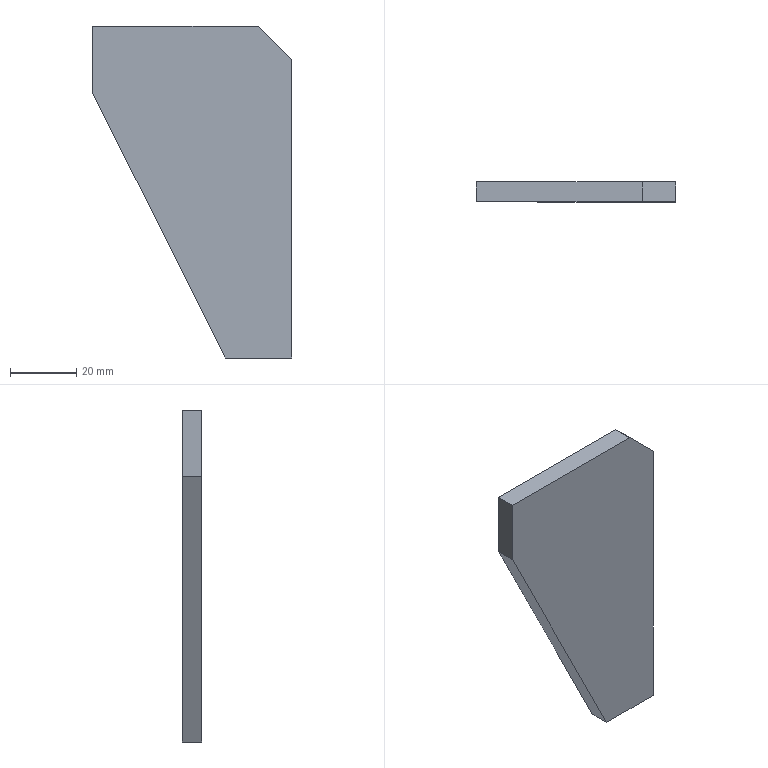Component | SolidWorks | JHK-B1004Stiffener-3 | 1 solid | 8 faces | box 60 x 6 x 100 mm | volume 26100 mm3 | plane 8 | material Q235A
build123d program:
from build123d import *

# Parameters (mm, degrees)
BOSS_EXTRUDE1_DEPTH = 3
CHAMFER1_SIZE       = 10


with BuildPart() as part:
    # Sketch1 → Boss-Extrude1 (new, symmetric)
    with BuildSketch(Plane(origin=(0, 0, 0), x_dir=(0, 0, -1), z_dir=(0, 1, 0))):
        Polygon((0, 60), (0, 0), (100, 0), (100, 20), (20, 60), align=None)
    extrude(amount=BOSS_EXTRUDE1_DEPTH, both=True)

    # Chamfer1
    chamfer1_edges = [part.edges().sort_by_distance(p)[0] for p in [
        (0, 0, 0),
    ]]
    chamfer(chamfer1_edges, length=CHAMFER1_SIZE)


solid = part.part

# Placed as in the assembly
solid = solid.moved(Location((270, -125, -261), (0, 0, 0)))
STEP:
#1=COLOUR_RGB('',0.7922,0.8196,0.9333);
#2=FILL_AREA_STYLE_COLOUR('',#1);
#3=FILL_AREA_STYLE('',(#2));
#4=SURFACE_STYLE_FILL_AREA(#3);
#5=SURFACE_SIDE_STYLE('',(#4));
#6=SURFACE_STYLE_USAGE(.BOTH.,#5);
#7=PRESENTATION_STYLE_ASSIGNMENT((#6));
#8=CARTESIAN_POINT('',(10.63,-4.803,-10.669));
#9=VERTEX_POINT('',#8);
#10=CARTESIAN_POINT('',(10.63,-4.803,-14.213));
#11=VERTEX_POINT('',#10);
#12=CARTESIAN_POINT('',(10.63,-4.803,-10.276));
#13=DIRECTION('',(0.,0.,-1.));
#14=VECTOR('',#13,39.37);
#15=LINE('',#12,#14);
#16=EDGE_CURVE('',#9,#11,#15,.T.);
#17=ORIENTED_EDGE('',*,*,#16,.F.);
#18=CARTESIAN_POINT('',(10.63,-5.039,-10.669));
#19=VERTEX_POINT('',#18);
#20=CARTESIAN_POINT('',(10.63,-4.803,-10.669));
#21=DIRECTION('',(0.,-1.,0.));
#22=VECTOR('',#21,39.37);
#23=LINE('',#20,#22);
#24=EDGE_CURVE('',#9,#19,#23,.T.);
#25=ORIENTED_EDGE('',*,*,#24,.T.);
#26=CARTESIAN_POINT('',(10.63,-5.039,-14.213));
#27=VERTEX_POINT('',#26);
#28=CARTESIAN_POINT('',(10.63,-5.039,-10.276));
#29=DIRECTION('',(0.,0.,-1.));
#30=VECTOR('',#29,39.37);
#31=LINE('',#28,#30);
#32=EDGE_CURVE('',#19,#27,#31,.T.);
#33=ORIENTED_EDGE('',*,*,#32,.T.);
#34=CARTESIAN_POINT('',(10.63,-4.803,-14.213));
#35=DIRECTION('',(0.,-1.,0.));
#36=VECTOR('',#35,39.37);
#37=LINE('',#34,#36);
#38=EDGE_CURVE('',#11,#27,#37,.T.);
#39=ORIENTED_EDGE('',*,*,#38,.F.);
#40=EDGE_LOOP('',(#17,#25,#33,#39));
#41=FACE_OUTER_BOUND('',#40,.T.);
#42=CARTESIAN_POINT('',(10.63,-4.803,-10.276));
#43=DIRECTION('',(-1.,0.,0.));
#44=DIRECTION('',(0.,0.,1.));
#45=AXIS2_PLACEMENT_3D('',#42,#43,#44);
#46=PLANE('',#45);
#47=ADVANCED_FACE('',(#41),#46,.F.);
#48=CARTESIAN_POINT('',(9.843,-5.039,-14.213));
#49=VERTEX_POINT('',#48);
#50=CARTESIAN_POINT('',(10.63,-5.039,-14.213));
#51=DIRECTION('',(-1.,0.,0.));
#52=VECTOR('',#51,39.37);
#53=LINE('',#50,#52);
#54=EDGE_CURVE('',#27,#49,#53,.T.);
#55=ORIENTED_EDGE('',*,*,#54,.T.);
#56=CARTESIAN_POINT('',(9.843,-4.803,-14.213));
#57=VERTEX_POINT('',#56);
#58=CARTESIAN_POINT('',(9.843,-4.803,-14.213));
#59=DIRECTION('',(0.,-1.,0.));
#60=VECTOR('',#59,39.37);
#61=LINE('',#58,#60);
#62=EDGE_CURVE('',#57,#49,#61,.T.);
#63=ORIENTED_EDGE('',*,*,#62,.F.);
#64=CARTESIAN_POINT('',(10.63,-4.803,-14.213));
#65=DIRECTION('',(-1.,0.,0.));
#66=VECTOR('',#65,39.37);
#67=LINE('',#64,#66);
#68=EDGE_CURVE('',#11,#57,#67,.T.);
#69=ORIENTED_EDGE('',*,*,#68,.F.);
#70=ORIENTED_EDGE('',*,*,#38,.T.);
#71=EDGE_LOOP('',(#55,#63,#69,#70));
#72=FACE_OUTER_BOUND('',#71,.T.);
#73=CARTESIAN_POINT('',(10.63,-4.803,-14.213));
#74=DIRECTION('',(0.,0.,1.));
#75=DIRECTION('',(1.,0.,0.));
#76=AXIS2_PLACEMENT_3D('',#73,#74,#75);
#77=PLANE('',#76);
#78=ADVANCED_FACE('',(#72),#77,.F.);
#79=CARTESIAN_POINT('',(8.268,-5.039,-11.063));
#80=VERTEX_POINT('',#79);
#81=CARTESIAN_POINT('',(9.843,-5.039,-14.213));
#82=DIRECTION('',(-0.4472,0.,0.8944));
#83=VECTOR('',#82,39.37);
#84=LINE('',#81,#83);
#85=EDGE_CURVE('',#49,#80,#84,.T.);
#86=ORIENTED_EDGE('',*,*,#85,.T.);
#87=CARTESIAN_POINT('',(8.268,-4.803,-11.063));
#88=VERTEX_POINT('',#87);
#89=CARTESIAN_POINT('',(8.268,-4.803,-11.063));
#90=DIRECTION('',(0.,-1.,0.));
#91=VECTOR('',#90,39.37);
#92=LINE('',#89,#91);
#93=EDGE_CURVE('',#88,#80,#92,.T.);
#94=ORIENTED_EDGE('',*,*,#93,.F.);
#95=CARTESIAN_POINT('',(9.843,-4.803,-14.213));
#96=DIRECTION('',(-0.4472,0.,0.8944));
#97=VECTOR('',#96,39.37);
#98=LINE('',#95,#97);
#99=EDGE_CURVE('',#57,#88,#98,.T.);
#100=ORIENTED_EDGE('',*,*,#99,.F.);
#101=ORIENTED_EDGE('',*,*,#62,.T.);
#102=EDGE_LOOP('',(#86,#94,#100,#101));
#103=FACE_OUTER_BOUND('',#102,.T.);
#104=CARTESIAN_POINT('',(9.843,-4.803,-14.213));
#105=DIRECTION('',(0.8944,0.,0.4472));
#106=DIRECTION('',(0.4472,0.,-0.8944));
#107=AXIS2_PLACEMENT_3D('',#104,#105,#106);
#108=PLANE('',#107);
#109=ADVANCED_FACE('',(#103),#108,.F.);
#110=CARTESIAN_POINT('',(8.268,-5.039,-10.276));
#111=VERTEX_POINT('',#110);
#112=CARTESIAN_POINT('',(8.268,-5.039,-11.063));
#113=DIRECTION('',(0.,0.,1.));
#114=VECTOR('',#113,39.37);
#115=LINE('',#112,#114);
#116=EDGE_CURVE('',#80,#111,#115,.T.);
#117=ORIENTED_EDGE('',*,*,#116,.T.);
#118=CARTESIAN_POINT('',(8.268,-4.803,-10.276));
#119=VERTEX_POINT('',#118);
#120=CARTESIAN_POINT('',(8.268,-4.803,-10.276));
#121=DIRECTION('',(0.,-1.,0.));
#122=VECTOR('',#121,39.37);
#123=LINE('',#120,#122);
#124=EDGE_CURVE('',#119,#111,#123,.T.);
#125=ORIENTED_EDGE('',*,*,#124,.F.);
#126=CARTESIAN_POINT('',(8.268,-4.803,-11.063));
#127=DIRECTION('',(0.,0.,1.));
#128=VECTOR('',#127,39.37);
#129=LINE('',#126,#128);
#130=EDGE_CURVE('',#88,#119,#129,.T.);
#131=ORIENTED_EDGE('',*,*,#130,.F.);
#132=ORIENTED_EDGE('',*,*,#93,.T.);
#133=EDGE_LOOP('',(#117,#125,#131,#132));
#134=FACE_OUTER_BOUND('',#133,.T.);
#135=CARTESIAN_POINT('',(8.268,-4.803,-11.063));
#136=DIRECTION('',(1.,0.,0.));
#137=DIRECTION('',(0.,0.,-1.));
#138=AXIS2_PLACEMENT_3D('',#135,#136,#137);
#139=PLANE('',#138);
#140=ADVANCED_FACE('',(#134),#139,.F.);
#141=CARTESIAN_POINT('',(10.236,-5.039,-10.276));
#142=VERTEX_POINT('',#141);
#143=CARTESIAN_POINT('',(8.268,-5.039,-10.276));
#144=DIRECTION('',(1.,0.,-0.));
#145=VECTOR('',#144,39.37);
#146=LINE('',#143,#145);
#147=EDGE_CURVE('',#111,#142,#146,.T.);
#148=ORIENTED_EDGE('',*,*,#147,.T.);
#149=CARTESIAN_POINT('',(10.236,-4.803,-10.276));
#150=VERTEX_POINT('',#149);
#151=CARTESIAN_POINT('',(10.236,-4.803,-10.276));
#152=DIRECTION('',(0.,1.,0.));
#153=VECTOR('',#152,39.37);
#154=LINE('',#151,#153);
#155=EDGE_CURVE('',#142,#150,#154,.T.);
#156=ORIENTED_EDGE('',*,*,#155,.T.);
#157=CARTESIAN_POINT('',(8.268,-4.803,-10.276));
#158=DIRECTION('',(1.,0.,-0.));
#159=VECTOR('',#158,39.37);
#160=LINE('',#157,#159);
#161=EDGE_CURVE('',#119,#150,#160,.T.);
#162=ORIENTED_EDGE('',*,*,#161,.F.);
#163=ORIENTED_EDGE('',*,*,#124,.T.);
#164=EDGE_LOOP('',(#148,#156,#162,#163));
#165=FACE_OUTER_BOUND('',#164,.T.);
#166=CARTESIAN_POINT('',(8.268,-4.803,-10.276));
#167=DIRECTION('',(-0.,0.,-1.));
#168=DIRECTION('',(-1.,0.,0.));
#169=AXIS2_PLACEMENT_3D('',#166,#167,#168);
#170=PLANE('',#169);
#171=ADVANCED_FACE('',(#165),#170,.F.);
#172=ORIENTED_EDGE('',*,*,#161,.T.);
#173=CARTESIAN_POINT('',(10.433,-4.803,-10.472));
#174=DIRECTION('',(0.7071,0.,-0.7071));
#175=VECTOR('',#174,39.37);
#176=LINE('',#173,#175);
#177=EDGE_CURVE('',#150,#9,#176,.T.);
#178=ORIENTED_EDGE('',*,*,#177,.T.);
#179=ORIENTED_EDGE('',*,*,#16,.T.);
#180=ORIENTED_EDGE('',*,*,#68,.T.);
#181=ORIENTED_EDGE('',*,*,#99,.T.);
#182=ORIENTED_EDGE('',*,*,#130,.T.);
#183=EDGE_LOOP('',(#172,#178,#179,#180,#181,#182));
#184=FACE_OUTER_BOUND('',#183,.T.);
#185=CARTESIAN_POINT('',(10.63,-4.803,-10.276));
#186=DIRECTION('',(0.,1.,0.));
#187=DIRECTION('',(0.,0.,1.));
#188=AXIS2_PLACEMENT_3D('',#185,#186,#187);
#189=PLANE('',#188);
#190=ADVANCED_FACE('',(#184),#189,.T.);
#191=ORIENTED_EDGE('',*,*,#32,.F.);
#192=CARTESIAN_POINT('',(10.63,-5.039,-10.669));
#193=DIRECTION('',(-0.7071,0.,0.7071));
#194=VECTOR('',#193,39.37);
#195=LINE('',#192,#194);
#196=EDGE_CURVE('',#19,#142,#195,.T.);
#197=ORIENTED_EDGE('',*,*,#196,.T.);
#198=ORIENTED_EDGE('',*,*,#147,.F.);
#199=ORIENTED_EDGE('',*,*,#116,.F.);
#200=ORIENTED_EDGE('',*,*,#85,.F.);
#201=ORIENTED_EDGE('',*,*,#54,.F.);
#202=EDGE_LOOP('',(#191,#197,#198,#199,#200,#201));
#203=FACE_OUTER_BOUND('',#202,.T.);
#204=CARTESIAN_POINT('',(10.63,-5.039,-10.276));
#205=DIRECTION('',(0.,1.,0.));
#206=DIRECTION('',(0.,0.,1.));
#207=AXIS2_PLACEMENT_3D('',#204,#205,#206);
#208=PLANE('',#207);
#209=ADVANCED_FACE('',(#203),#208,.F.);
#210=ORIENTED_EDGE('',*,*,#177,.F.);
#211=ORIENTED_EDGE('',*,*,#155,.F.);
#212=ORIENTED_EDGE('',*,*,#196,.F.);
#213=ORIENTED_EDGE('',*,*,#24,.F.);
#214=EDGE_LOOP('',(#210,#211,#212,#213));
#215=FACE_OUTER_BOUND('',#214,.T.);
#216=CARTESIAN_POINT('',(10.63,-4.803,-10.669));
#217=DIRECTION('',(-0.7071,0.,-0.7071));
#218=DIRECTION('',(0.,-1.,0.));
#219=AXIS2_PLACEMENT_3D('',#216,#217,#218);
#220=PLANE('',#219);
#221=ADVANCED_FACE('',(#215),#220,.F.);
#222=CLOSED_SHELL('',(#47,#78,#109,#140,#171,#190,#209,#221));
#223=MANIFOLD_SOLID_BREP('',#222);
#224=STYLED_ITEM('',(#7),#223);
#225=(LENGTH_UNIT()NAMED_UNIT(*)SI_UNIT($,.METRE.));
#226=LENGTH_MEASURE_WITH_UNIT(LENGTH_MEASURE(0.0254),#225);
#227=DIMENSIONAL_EXPONENTS(1.,0.,0.,0.,0.,0.,0.);
#228=(CONVERSION_BASED_UNIT('',#226)LENGTH_UNIT()NAMED_UNIT(#227));
#229=UNCERTAINTY_MEASURE_WITH_UNIT(LENGTH_MEASURE(0.00001),#228,'','');
#230=(NAMED_UNIT(*)PLANE_ANGLE_UNIT()SI_UNIT($,.RADIAN.));
#231=(NAMED_UNIT(*)SI_UNIT($,.STERADIAN.)SOLID_ANGLE_UNIT());
#232=(GEOMETRIC_REPRESENTATION_CONTEXT(3)GLOBAL_UNCERTAINTY_ASSIGNED_CONTEXT((#229))GLOBAL_UNIT_ASSIGNED_CONTEXT((#228,#230,#231))REPRESENTATION_CONTEXT('',''));
#233=MECHANICAL_DESIGN_GEOMETRIC_PRESENTATION_REPRESENTATION('',(#224),#232);
#234=CARTESIAN_POINT('',(0.,0.,0.));
#235=DIRECTION('',(0.,0.,1.));
#236=DIRECTION('',(1.,0.,0.));
#237=AXIS2_PLACEMENT_3D('',#234,#235,#236);
#238=(LENGTH_UNIT()NAMED_UNIT(*)SI_UNIT($,.METRE.));
#239=LENGTH_MEASURE_WITH_UNIT(LENGTH_MEASURE(0.0254),#238);
#240=DIMENSIONAL_EXPONENTS(1.,0.,0.,0.,0.,0.,0.);
#241=(CONVERSION_BASED_UNIT('',#239)LENGTH_UNIT()NAMED_UNIT(#240));
#242=UNCERTAINTY_MEASURE_WITH_UNIT(LENGTH_MEASURE(0.00001),#241,'','');
#243=(NAMED_UNIT(*)PLANE_ANGLE_UNIT()SI_UNIT($,.RADIAN.));
#244=(NAMED_UNIT(*)SI_UNIT($,.STERADIAN.)SOLID_ANGLE_UNIT());
#245=(GEOMETRIC_REPRESENTATION_CONTEXT(3)GLOBAL_UNCERTAINTY_ASSIGNED_CONTEXT((#242))GLOBAL_UNIT_ASSIGNED_CONTEXT((#241,#243,#244))REPRESENTATION_CONTEXT('',''));
#246=ADVANCED_BREP_SHAPE_REPRESENTATION('',(#223,#237),#245);
#247=PRESENTATION_LAYER_ASSIGNMENT('','',(#224));